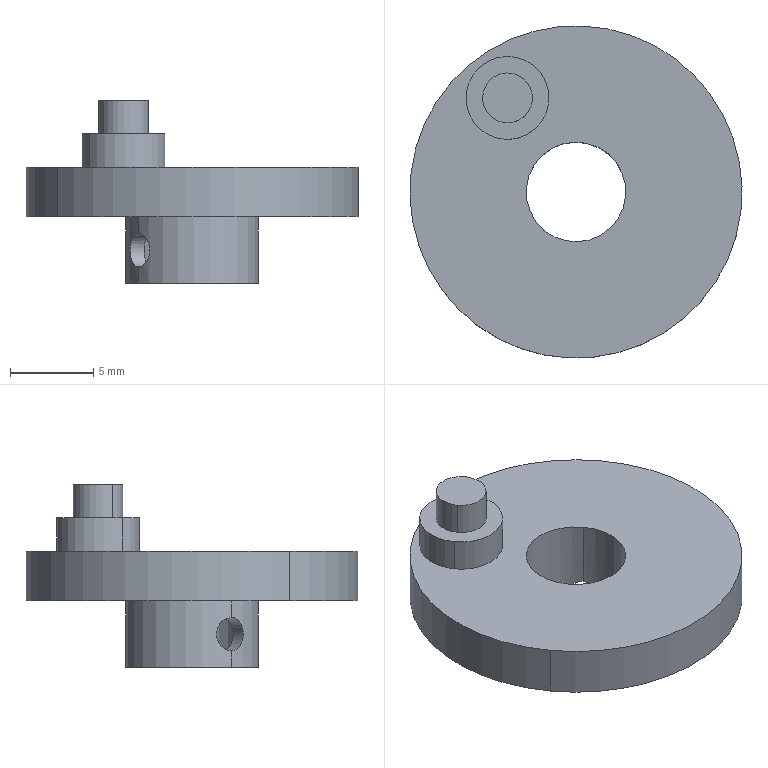Component | SolidWorks | 10-1 | 1 solid | 19 faces | box 20 x 20 x 11 mm | volume 993 mm3 | cylinder 14 | plane 5 | commonest cylinder face diameters 2 x4 8 x2 6 x2 3 x2 5 x2 20 x2
build123d program:
from build123d import *

# Parameters (mm, degrees)
SKETCH1_R           = 10
BOSS_EXTRUDE1_DEPTH = 3
SKETCH2_R           = 2.5
BOSS_EXTRUDE2_DEPTH = 2
SKETCH3_R           = 1.5
BOSS_EXTRUDE3_DEPTH = 2
SKETCH4_R           = 3
CUT_EXTRUDE1_DEPTH  = 24
BOSS_EXTRUDE4_START = 4
SKETCH5_R           = 4
SKETCH5_R_2         = 3
BOSS_EXTRUDE4_DEPTH = 4
SKETCH6_R           = 1
CUT_EXTRUDE2_DEPTH  = 5


with BuildPart() as part:
    # Sketch1 → Boss-Extrude1 (new body)
    with BuildSketch(Plane.XY):
        Circle(SKETCH1_R)
    extrude(amount=BOSS_EXTRUDE1_DEPTH)

    # Sketch2 → Boss-Extrude2 (add)
    with BuildSketch(Plane.XY.offset(3)):
        with Locations((0, 7)):
            Circle(SKETCH2_R)
    extrude(amount=BOSS_EXTRUDE2_DEPTH)

    # Sketch3 → Boss-Extrude3 (add)
    with BuildSketch(Plane.XY.offset(5)):
        with Locations((0, 7)):
            Circle(SKETCH3_R)
    extrude(amount=BOSS_EXTRUDE3_DEPTH)

    # Sketch4 → Cut-Extrude1 (cut)
    with BuildSketch(Plane(origin=(0, 0, 0), x_dir=(-1, 0, 0), z_dir=(0, 0, -1))):
        Circle(SKETCH4_R)
    extrude(amount=-CUT_EXTRUDE1_DEPTH, mode=Mode.SUBTRACT)

    # Sketch5 → Boss-Extrude4 (add)
    with BuildSketch(Plane(origin=(0, 0, 0), x_dir=(-1, 0, 0), z_dir=(0, 0, -1)).offset(BOSS_EXTRUDE4_START)):
        with Locations(Location((0, 0, 0), (0, 0, 180))):
            Circle(SKETCH5_R)
        Circle(SKETCH5_R_2, mode=Mode.SUBTRACT)
    extrude(amount=-BOSS_EXTRUDE4_DEPTH)

    # Sketch6 → Cut-Extrude2 (cut, symmetric)
    with BuildSketch(Plane(origin=(0, 0, 0), x_dir=(0, 0, -1), z_dir=(1, 0, 0))):
        with Locations((2, 0)):
            Circle(SKETCH6_R)
    extrude(amount=CUT_EXTRUDE2_DEPTH, both=True, mode=Mode.SUBTRACT)


solid = part.part

# Placed as in the assembly
solid = solid.moved(Location((69.329, 7.034, 22.938), (0, 0, 36.07)))
STEP:
#1=COLOUR_RGB('',0.7922,0.8196,0.9333);
#2=FILL_AREA_STYLE_COLOUR('',#1);
#3=FILL_AREA_STYLE('',(#2));
#4=SURFACE_STYLE_FILL_AREA(#3);
#5=SURFACE_SIDE_STYLE('',(#4));
#6=SURFACE_STYLE_USAGE(.BOTH.,#5);
#7=PRESENTATION_STYLE_ASSIGNMENT((#6));
#8=CARTESIAN_POINT('',(2.825,0.3465,0.8637));
#9=VERTEX_POINT('',#8);
#10=CARTESIAN_POINT('',(2.825,0.3465,0.785));
#11=VERTEX_POINT('',#10);
#12=CARTESIAN_POINT('',(2.825,0.3465,0.8637));
#13=CARTESIAN_POINT('',(2.828,0.3423,0.8637));
#14=CARTESIAN_POINT('',(2.831,0.3379,0.8627));
#15=CARTESIAN_POINT('',(2.835,0.3295,0.8587));
#16=CARTESIAN_POINT('',(2.837,0.3255,0.8558));
#17=CARTESIAN_POINT('',(2.84,0.3185,0.8485));
#18=CARTESIAN_POINT('',(2.841,0.3157,0.8442));
#19=CARTESIAN_POINT('',(2.842,0.3117,0.8347));
#20=CARTESIAN_POINT('',(2.843,0.3107,0.8295));
#21=CARTESIAN_POINT('',(2.843,0.3107,0.8191));
#22=CARTESIAN_POINT('',(2.842,0.3117,0.8139));
#23=CARTESIAN_POINT('',(2.841,0.3157,0.8045));
#24=CARTESIAN_POINT('',(2.84,0.3186,0.8001));
#25=CARTESIAN_POINT('',(2.837,0.3254,0.7929));
#26=CARTESIAN_POINT('',(2.835,0.3294,0.79));
#27=CARTESIAN_POINT('',(2.831,0.3379,0.786));
#28=CARTESIAN_POINT('',(2.828,0.3422,0.785));
#29=CARTESIAN_POINT('',(2.825,0.3465,0.785));
#30=B_SPLINE_CURVE_WITH_KNOTS('',3,(#12,#13,#14,#15,#16,#17,#18,#19,#20,#21,#22,#23,#24,#25,#26,#27,#28,#29),.UNSPECIFIED.,.F.,.F.,(4,2,2,2,2,2,2,2,4),(0.003149,0.003543,0.003936,0.00433,0.004723,0.005117,0.00551,0.005904,0.006298),.UNSPECIFIED.);
#31=EDGE_CURVE('',#9,#11,#30,.T.);
#32=ORIENTED_EDGE('',*,*,#31,.F.);
#33=CARTESIAN_POINT('',(2.857,0.3696,0.8637));
#34=VERTEX_POINT('',#33);
#35=CARTESIAN_POINT('',(2.57,0.161,0.8637));
#36=DIRECTION('',(0.8083,0.5888,-0.));
#37=VECTOR('',#36,39.37);
#38=LINE('',#35,#37);
#39=EDGE_CURVE('',#9,#34,#38,.T.);
#40=ORIENTED_EDGE('',*,*,#39,.T.);
#41=CARTESIAN_POINT('',(2.857,0.3696,0.785));
#42=VERTEX_POINT('',#41);
#43=CARTESIAN_POINT('',(2.857,0.3696,0.785));
#44=CARTESIAN_POINT('',(2.86,0.3654,0.785));
#45=CARTESIAN_POINT('',(2.863,0.3611,0.786));
#46=CARTESIAN_POINT('',(2.868,0.3529,0.79));
#47=CARTESIAN_POINT('',(2.87,0.349,0.7929));
#48=CARTESIAN_POINT('',(2.873,0.3424,0.8001));
#49=CARTESIAN_POINT('',(2.874,0.3396,0.8045));
#50=CARTESIAN_POINT('',(2.876,0.3359,0.814));
#51=CARTESIAN_POINT('',(2.876,0.3349,0.8192));
#52=CARTESIAN_POINT('',(2.876,0.3349,0.8295));
#53=CARTESIAN_POINT('',(2.876,0.3359,0.8346));
#54=CARTESIAN_POINT('',(2.874,0.3396,0.8442));
#55=CARTESIAN_POINT('',(2.873,0.3424,0.8485));
#56=CARTESIAN_POINT('',(2.87,0.349,0.8558));
#57=CARTESIAN_POINT('',(2.868,0.3529,0.8587));
#58=CARTESIAN_POINT('',(2.863,0.3611,0.8627));
#59=CARTESIAN_POINT('',(2.86,0.3655,0.8637));
#60=CARTESIAN_POINT('',(2.857,0.3696,0.8637));
#61=B_SPLINE_CURVE_WITH_KNOTS('',3,(#43,#44,#45,#46,#47,#48,#49,#50,#51,#52,#53,#54,#55,#56,#57,#58,#59,#60),.UNSPECIFIED.,.F.,.F.,(4,2,2,2,2,2,2,2,4),(0.,0.0003924,0.0007847,0.001177,0.001569,0.001962,0.002354,0.002747,0.003139),.UNSPECIFIED.);
#62=EDGE_CURVE('',#42,#34,#61,.T.);
#63=ORIENTED_EDGE('',*,*,#62,.F.);
#64=CARTESIAN_POINT('',(2.57,0.161,0.785));
#65=DIRECTION('',(0.8083,0.5888,-0.));
#66=VECTOR('',#65,39.37);
#67=LINE('',#64,#66);
#68=EDGE_CURVE('',#11,#42,#67,.T.);
#69=ORIENTED_EDGE('',*,*,#68,.F.);
#70=EDGE_LOOP('',(#32,#40,#63,#69));
#71=FACE_OUTER_BOUND('',#70,.T.);
#72=CARTESIAN_POINT('',(2.57,0.161,0.8243));
#73=DIRECTION('',(0.8083,0.5888,-0.));
#74=DIRECTION('',(0.,-0.,-1.));
#75=AXIS2_PLACEMENT_3D('',#72,#73,#74);
#76=CYLINDRICAL_SURFACE('',#75,0.03937);
#77=ADVANCED_FACE('',(#71),#76,.F.);
#78=CARTESIAN_POINT('',(2.602,0.1842,0.8637));
#79=VERTEX_POINT('',#78);
#80=CARTESIAN_POINT('',(2.602,0.1842,0.785));
#81=VERTEX_POINT('',#80);
#82=CARTESIAN_POINT('',(2.602,0.1842,0.8637));
#83=CARTESIAN_POINT('',(2.605,0.18,0.8637));
#84=CARTESIAN_POINT('',(2.609,0.176,0.8627));
#85=CARTESIAN_POINT('',(2.615,0.1689,0.8587));
#86=CARTESIAN_POINT('',(2.618,0.1657,0.8558));
#87=CARTESIAN_POINT('',(2.623,0.1606,0.8486));
#88=CARTESIAN_POINT('',(2.626,0.1587,0.8442));
#89=CARTESIAN_POINT('',(2.629,0.156,0.8347));
#90=CARTESIAN_POINT('',(2.629,0.1553,0.8295));
#91=CARTESIAN_POINT('',(2.629,0.1553,0.8192));
#92=CARTESIAN_POINT('',(2.629,0.156,0.814));
#93=CARTESIAN_POINT('',(2.626,0.1586,0.8045));
#94=CARTESIAN_POINT('',(2.623,0.1606,0.8001));
#95=CARTESIAN_POINT('',(2.618,0.1657,0.7929));
#96=CARTESIAN_POINT('',(2.615,0.1688,0.79));
#97=CARTESIAN_POINT('',(2.609,0.176,0.786));
#98=CARTESIAN_POINT('',(2.605,0.18,0.785));
#99=CARTESIAN_POINT('',(2.602,0.1842,0.785));
#100=B_SPLINE_CURVE_WITH_KNOTS('',3,(#82,#83,#84,#85,#86,#87,#88,#89,#90,#91,#92,#93,#94,#95,#96,#97,#98,#99),.UNSPECIFIED.,.F.,.F.,(4,2,2,2,2,2,2,2,4),(0.003139,0.003531,0.003923,0.004316,0.004708,0.0051,0.005493,0.005885,0.006277),.UNSPECIFIED.);
#101=EDGE_CURVE('',#79,#81,#100,.T.);
#102=ORIENTED_EDGE('',*,*,#101,.F.);
#103=CARTESIAN_POINT('',(2.634,0.2074,0.8637));
#104=VERTEX_POINT('',#103);
#105=CARTESIAN_POINT('',(2.57,0.161,0.8637));
#106=DIRECTION('',(0.8083,0.5888,-0.));
#107=VECTOR('',#106,39.37);
#108=LINE('',#105,#107);
#109=EDGE_CURVE('',#79,#104,#108,.T.);
#110=ORIENTED_EDGE('',*,*,#109,.T.);
#111=CARTESIAN_POINT('',(2.634,0.2074,0.785));
#112=VERTEX_POINT('',#111);
#113=CARTESIAN_POINT('',(2.634,0.2074,0.785));
#114=CARTESIAN_POINT('',(2.637,0.2032,0.785));
#115=CARTESIAN_POINT('',(2.64,0.1992,0.786));
#116=CARTESIAN_POINT('',(2.647,0.1923,0.79));
#117=CARTESIAN_POINT('',(2.65,0.1893,0.7929));
#118=CARTESIAN_POINT('',(2.656,0.1844,0.8001));
#119=CARTESIAN_POINT('',(2.658,0.1826,0.8044));
#120=CARTESIAN_POINT('',(2.662,0.1802,0.814));
#121=CARTESIAN_POINT('',(2.663,0.1795,0.8192));
#122=CARTESIAN_POINT('',(2.663,0.1795,0.8295));
#123=CARTESIAN_POINT('',(2.662,0.1802,0.8347));
#124=CARTESIAN_POINT('',(2.658,0.1826,0.8442));
#125=CARTESIAN_POINT('',(2.656,0.1844,0.8486));
#126=CARTESIAN_POINT('',(2.65,0.1892,0.8558));
#127=CARTESIAN_POINT('',(2.647,0.1922,0.8587));
#128=CARTESIAN_POINT('',(2.64,0.1992,0.8627));
#129=CARTESIAN_POINT('',(2.637,0.2032,0.8637));
#130=CARTESIAN_POINT('',(2.634,0.2074,0.8637));
#131=B_SPLINE_CURVE_WITH_KNOTS('',3,(#113,#114,#115,#116,#117,#118,#119,#120,#121,#122,#123,#124,#125,#126,#127,#128,#129,#130),.UNSPECIFIED.,.F.,.F.,(4,2,2,2,2,2,2,2,4),(0.003149,0.003543,0.003936,0.00433,0.004723,0.005117,0.00551,0.005904,0.006298),.UNSPECIFIED.);
#132=EDGE_CURVE('',#112,#104,#131,.T.);
#133=ORIENTED_EDGE('',*,*,#132,.F.);
#134=CARTESIAN_POINT('',(2.57,0.161,0.785));
#135=DIRECTION('',(0.8083,0.5888,-0.));
#136=VECTOR('',#135,39.37);
#137=LINE('',#134,#136);
#138=EDGE_CURVE('',#81,#112,#137,.T.);
#139=ORIENTED_EDGE('',*,*,#138,.F.);
#140=EDGE_LOOP('',(#102,#110,#133,#139));
#141=FACE_OUTER_BOUND('',#140,.T.);
#142=CARTESIAN_POINT('',(2.57,0.161,0.8243));
#143=DIRECTION('',(0.8083,0.5888,-0.));
#144=DIRECTION('',(0.,-0.,-1.));
#145=AXIS2_PLACEMENT_3D('',#142,#143,#144);
#146=CYLINDRICAL_SURFACE('',#145,0.03937);
#147=ADVANCED_FACE('',(#141),#146,.F.);
#148=CARTESIAN_POINT('',(2.602,0.1842,0.7456));
#149=VERTEX_POINT('',#148);
#150=CARTESIAN_POINT('',(2.857,0.3696,0.7456));
#151=VERTEX_POINT('',#150);
#152=CARTESIAN_POINT('',(2.73,0.2769,0.7456));
#153=DIRECTION('',(-0.,-0.,-1.));
#154=DIRECTION('',(-0.8083,-0.5888,0.));
#155=AXIS2_PLACEMENT_3D('',#152,#153,#154);
#156=CIRCLE('',#155,0.1575);
#157=EDGE_CURVE('',#149,#151,#156,.T.);
#158=ORIENTED_EDGE('',*,*,#157,.F.);
#159=CARTESIAN_POINT('',(2.602,0.1842,0.7456));
#160=DIRECTION('',(0.,0.,1.));
#161=VECTOR('',#160,39.37);
#162=LINE('',#159,#161);
#163=EDGE_CURVE('',#149,#81,#162,.T.);
#164=ORIENTED_EDGE('',*,*,#163,.T.);
#165=CARTESIAN_POINT('',(2.602,0.1842,0.785));
#166=CARTESIAN_POINT('',(2.599,0.1884,0.785));
#167=CARTESIAN_POINT('',(2.596,0.1927,0.786));
#168=CARTESIAN_POINT('',(2.591,0.201,0.79));
#169=CARTESIAN_POINT('',(2.589,0.2049,0.7929));
#170=CARTESIAN_POINT('',(2.586,0.2115,0.8001));
#171=CARTESIAN_POINT('',(2.585,0.2142,0.8045));
#172=CARTESIAN_POINT('',(2.583,0.218,0.814));
#173=CARTESIAN_POINT('',(2.583,0.219,0.8192));
#174=CARTESIAN_POINT('',(2.583,0.219,0.8295));
#175=CARTESIAN_POINT('',(2.583,0.218,0.8346));
#176=CARTESIAN_POINT('',(2.585,0.2142,0.8442));
#177=CARTESIAN_POINT('',(2.586,0.2115,0.8485));
#178=CARTESIAN_POINT('',(2.589,0.2048,0.8558));
#179=CARTESIAN_POINT('',(2.591,0.2009,0.8587));
#180=CARTESIAN_POINT('',(2.596,0.1927,0.8627));
#181=CARTESIAN_POINT('',(2.599,0.1884,0.8637));
#182=CARTESIAN_POINT('',(2.602,0.1842,0.8637));
#183=B_SPLINE_CURVE_WITH_KNOTS('',3,(#165,#166,#167,#168,#169,#170,#171,#172,#173,#174,#175,#176,#177,#178,#179,#180,#181,#182),.UNSPECIFIED.,.F.,.F.,(4,2,2,2,2,2,2,2,4),(0.,0.0003924,0.0007847,0.001177,0.001569,0.001962,0.002354,0.002747,0.003139),.UNSPECIFIED.);
#184=EDGE_CURVE('',#81,#79,#183,.T.);
#185=ORIENTED_EDGE('',*,*,#184,.T.);
#186=CARTESIAN_POINT('',(2.602,0.1842,0.9031));
#187=VERTEX_POINT('',#186);
#188=CARTESIAN_POINT('',(2.602,0.1842,0.7456));
#189=DIRECTION('',(0.,0.,1.));
#190=VECTOR('',#189,39.37);
#191=LINE('',#188,#190);
#192=EDGE_CURVE('',#79,#187,#191,.T.);
#193=ORIENTED_EDGE('',*,*,#192,.T.);
#194=CARTESIAN_POINT('',(2.857,0.3696,0.9031));
#195=VERTEX_POINT('',#194);
#196=CARTESIAN_POINT('',(2.73,0.2769,0.9031));
#197=DIRECTION('',(-0.,-0.,-1.));
#198=DIRECTION('',(0.8083,0.5888,-0.));
#199=AXIS2_PLACEMENT_3D('',#196,#197,#198);
#200=CIRCLE('',#199,0.1575);
#201=EDGE_CURVE('',#187,#195,#200,.T.);
#202=ORIENTED_EDGE('',*,*,#201,.T.);
#203=CARTESIAN_POINT('',(2.857,0.3696,0.7456));
#204=DIRECTION('',(0.,0.,1.));
#205=VECTOR('',#204,39.37);
#206=LINE('',#203,#205);
#207=EDGE_CURVE('',#34,#195,#206,.T.);
#208=ORIENTED_EDGE('',*,*,#207,.F.);
#209=CARTESIAN_POINT('',(2.857,0.3696,0.8637));
#210=CARTESIAN_POINT('',(2.854,0.3738,0.8637));
#211=CARTESIAN_POINT('',(2.85,0.3779,0.8627));
#212=CARTESIAN_POINT('',(2.844,0.385,0.8587));
#213=CARTESIAN_POINT('',(2.841,0.3881,0.8558));
#214=CARTESIAN_POINT('',(2.836,0.3932,0.8486));
#215=CARTESIAN_POINT('',(2.834,0.3952,0.8442));
#216=CARTESIAN_POINT('',(2.83,0.3979,0.8347));
#217=CARTESIAN_POINT('',(2.83,0.3985,0.8295));
#218=CARTESIAN_POINT('',(2.83,0.3985,0.8192));
#219=CARTESIAN_POINT('',(2.83,0.3979,0.814));
#220=CARTESIAN_POINT('',(2.833,0.3952,0.8045));
#221=CARTESIAN_POINT('',(2.836,0.3932,0.8001));
#222=CARTESIAN_POINT('',(2.841,0.3882,0.7929));
#223=CARTESIAN_POINT('',(2.844,0.385,0.79));
#224=CARTESIAN_POINT('',(2.85,0.3779,0.786));
#225=CARTESIAN_POINT('',(2.854,0.3739,0.785));
#226=CARTESIAN_POINT('',(2.857,0.3696,0.785));
#227=B_SPLINE_CURVE_WITH_KNOTS('',3,(#209,#210,#211,#212,#213,#214,#215,#216,#217,#218,#219,#220,#221,#222,#223,#224,#225,#226),.UNSPECIFIED.,.F.,.F.,(4,2,2,2,2,2,2,2,4),(0.003139,0.003531,0.003923,0.004316,0.004708,0.0051,0.005493,0.005885,0.006277),.UNSPECIFIED.);
#228=EDGE_CURVE('',#34,#42,#227,.T.);
#229=ORIENTED_EDGE('',*,*,#228,.T.);
#230=CARTESIAN_POINT('',(2.857,0.3696,0.7456));
#231=DIRECTION('',(0.,0.,1.));
#232=VECTOR('',#231,39.37);
#233=LINE('',#230,#232);
#234=EDGE_CURVE('',#151,#42,#233,.T.);
#235=ORIENTED_EDGE('',*,*,#234,.F.);
#236=EDGE_LOOP('',(#158,#164,#185,#193,#202,#208,#229,#235));
#237=FACE_OUTER_BOUND('',#236,.T.);
#238=CARTESIAN_POINT('',(2.73,0.2769,0.7456));
#239=DIRECTION('',(0.,0.,1.));
#240=DIRECTION('',(0.8083,0.5888,-0.));
#241=AXIS2_PLACEMENT_3D('',#238,#239,#240);
#242=CYLINDRICAL_SURFACE('',#241,0.1575);
#243=ADVANCED_FACE('',(#237),#242,.T.);
#244=CARTESIAN_POINT('',(2.634,0.2074,1.021));
#245=VERTEX_POINT('',#244);
#246=CARTESIAN_POINT('',(2.825,0.3465,1.021));
#247=VERTEX_POINT('',#246);
#248=CARTESIAN_POINT('',(2.73,0.2769,1.021));
#249=DIRECTION('',(0.,0.,1.));
#250=DIRECTION('',(0.8083,0.5888,-0.));
#251=AXIS2_PLACEMENT_3D('',#248,#249,#250);
#252=CIRCLE('',#251,0.1181);
#253=EDGE_CURVE('',#245,#247,#252,.T.);
#254=ORIENTED_EDGE('',*,*,#253,.T.);
#255=CARTESIAN_POINT('',(2.825,0.3465,1.848));
#256=DIRECTION('',(-0.,-0.,-1.));
#257=VECTOR('',#256,39.37);
#258=LINE('',#255,#257);
#259=EDGE_CURVE('',#247,#9,#258,.T.);
#260=ORIENTED_EDGE('',*,*,#259,.T.);
#261=ORIENTED_EDGE('',*,*,#31,.T.);
#262=CARTESIAN_POINT('',(2.825,0.3465,0.7456));
#263=VERTEX_POINT('',#262);
#264=CARTESIAN_POINT('',(2.825,0.3465,1.848));
#265=DIRECTION('',(-0.,-0.,-1.));
#266=VECTOR('',#265,39.37);
#267=LINE('',#264,#266);
#268=EDGE_CURVE('',#11,#263,#267,.T.);
#269=ORIENTED_EDGE('',*,*,#268,.T.);
#270=CARTESIAN_POINT('',(2.634,0.2074,0.7456));
#271=VERTEX_POINT('',#270);
#272=CARTESIAN_POINT('',(2.73,0.2769,0.7456));
#273=DIRECTION('',(-0.,-0.,-1.));
#274=DIRECTION('',(-0.8083,-0.5888,0.));
#275=AXIS2_PLACEMENT_3D('',#272,#273,#274);
#276=CIRCLE('',#275,0.1181);
#277=EDGE_CURVE('',#263,#271,#276,.T.);
#278=ORIENTED_EDGE('',*,*,#277,.T.);
#279=CARTESIAN_POINT('',(2.634,0.2074,1.848));
#280=DIRECTION('',(-0.,-0.,-1.));
#281=VECTOR('',#280,39.37);
#282=LINE('',#279,#281);
#283=EDGE_CURVE('',#112,#271,#282,.T.);
#284=ORIENTED_EDGE('',*,*,#283,.F.);
#285=ORIENTED_EDGE('',*,*,#132,.T.);
#286=CARTESIAN_POINT('',(2.634,0.2074,1.848));
#287=DIRECTION('',(-0.,-0.,-1.));
#288=VECTOR('',#287,39.37);
#289=LINE('',#286,#288);
#290=EDGE_CURVE('',#245,#104,#289,.T.);
#291=ORIENTED_EDGE('',*,*,#290,.F.);
#292=EDGE_LOOP('',(#254,#260,#261,#269,#278,#284,#285,#291));
#293=FACE_OUTER_BOUND('',#292,.T.);
#294=CARTESIAN_POINT('',(2.73,0.2769,1.848));
#295=DIRECTION('',(-0.,-0.,-1.));
#296=DIRECTION('',(-0.8083,-0.5888,0.));
#297=AXIS2_PLACEMENT_3D('',#294,#295,#296);
#298=CYLINDRICAL_SURFACE('',#297,0.1181);
#299=ADVANCED_FACE('',(#293),#298,.F.);
#300=CARTESIAN_POINT('',(2.615,0.5345,1.179));
#301=VERTEX_POINT('',#300);
#302=CARTESIAN_POINT('',(2.52,0.4649,1.179));
#303=VERTEX_POINT('',#302);
#304=CARTESIAN_POINT('',(2.567,0.4997,1.179));
#305=DIRECTION('',(0.,0.,1.));
#306=DIRECTION('',(0.8083,0.5888,-0.));
#307=AXIS2_PLACEMENT_3D('',#304,#305,#306);
#308=CIRCLE('',#307,0.05906);
#309=EDGE_CURVE('',#301,#303,#308,.T.);
#310=ORIENTED_EDGE('',*,*,#309,.F.);
#311=CARTESIAN_POINT('',(2.615,0.5345,1.1));
#312=VERTEX_POINT('',#311);
#313=CARTESIAN_POINT('',(2.615,0.5345,1.179));
#314=DIRECTION('',(-0.,-0.,-1.));
#315=VECTOR('',#314,39.37);
#316=LINE('',#313,#315);
#317=EDGE_CURVE('',#301,#312,#316,.T.);
#318=ORIENTED_EDGE('',*,*,#317,.T.);
#319=CARTESIAN_POINT('',(2.52,0.4649,1.1));
#320=VERTEX_POINT('',#319);
#321=CARTESIAN_POINT('',(2.567,0.4997,1.1));
#322=DIRECTION('',(0.,0.,1.));
#323=DIRECTION('',(0.8083,0.5888,-0.));
#324=AXIS2_PLACEMENT_3D('',#321,#322,#323);
#325=CIRCLE('',#324,0.05906);
#326=EDGE_CURVE('',#312,#320,#325,.T.);
#327=ORIENTED_EDGE('',*,*,#326,.T.);
#328=CARTESIAN_POINT('',(2.52,0.4649,1.179));
#329=DIRECTION('',(-0.,-0.,-1.));
#330=VECTOR('',#329,39.37);
#331=LINE('',#328,#330);
#332=EDGE_CURVE('',#303,#320,#331,.T.);
#333=ORIENTED_EDGE('',*,*,#332,.F.);
#334=EDGE_LOOP('',(#310,#318,#327,#333));
#335=FACE_OUTER_BOUND('',#334,.T.);
#336=CARTESIAN_POINT('',(2.567,0.4997,1.179));
#337=DIRECTION('',(-0.,-0.,-1.));
#338=DIRECTION('',(-0.8083,-0.5888,0.));
#339=AXIS2_PLACEMENT_3D('',#336,#337,#338);
#340=CYLINDRICAL_SURFACE('',#339,0.05906);
#341=ADVANCED_FACE('',(#335),#340,.T.);
#342=CARTESIAN_POINT('',(2.647,0.5576,1.1));
#343=VERTEX_POINT('',#342);
#344=CARTESIAN_POINT('',(2.488,0.4417,1.1));
#345=VERTEX_POINT('',#344);
#346=CARTESIAN_POINT('',(2.567,0.4997,1.1));
#347=DIRECTION('',(0.,0.,1.));
#348=DIRECTION('',(0.8083,0.5888,-0.));
#349=AXIS2_PLACEMENT_3D('',#346,#347,#348);
#350=CIRCLE('',#349,0.09843);
#351=EDGE_CURVE('',#343,#345,#350,.T.);
#352=ORIENTED_EDGE('',*,*,#351,.F.);
#353=CARTESIAN_POINT('',(2.647,0.5576,1.021));
#354=VERTEX_POINT('',#353);
#355=CARTESIAN_POINT('',(2.647,0.5576,1.1));
#356=DIRECTION('',(-0.,-0.,-1.));
#357=VECTOR('',#356,39.37);
#358=LINE('',#355,#357);
#359=EDGE_CURVE('',#343,#354,#358,.T.);
#360=ORIENTED_EDGE('',*,*,#359,.T.);
#361=CARTESIAN_POINT('',(2.488,0.4417,1.021));
#362=VERTEX_POINT('',#361);
#363=CARTESIAN_POINT('',(2.567,0.4997,1.021));
#364=DIRECTION('',(0.,0.,1.));
#365=DIRECTION('',(0.8083,0.5888,-0.));
#366=AXIS2_PLACEMENT_3D('',#363,#364,#365);
#367=CIRCLE('',#366,0.09843);
#368=EDGE_CURVE('',#354,#362,#367,.T.);
#369=ORIENTED_EDGE('',*,*,#368,.T.);
#370=CARTESIAN_POINT('',(2.488,0.4417,1.1));
#371=DIRECTION('',(-0.,-0.,-1.));
#372=VECTOR('',#371,39.37);
#373=LINE('',#370,#372);
#374=EDGE_CURVE('',#345,#362,#373,.T.);
#375=ORIENTED_EDGE('',*,*,#374,.F.);
#376=EDGE_LOOP('',(#352,#360,#369,#375));
#377=FACE_OUTER_BOUND('',#376,.T.);
#378=CARTESIAN_POINT('',(2.567,0.4997,1.1));
#379=DIRECTION('',(-0.,-0.,-1.));
#380=DIRECTION('',(-0.8083,-0.5888,0.));
#381=AXIS2_PLACEMENT_3D('',#378,#379,#380);
#382=CYLINDRICAL_SURFACE('',#381,0.09843);
#383=ADVANCED_FACE('',(#377),#382,.T.);
#384=CARTESIAN_POINT('',(3.048,0.5087,1.021));
#385=VERTEX_POINT('',#384);
#386=CARTESIAN_POINT('',(2.411,0.04513,1.021));
#387=VERTEX_POINT('',#386);
#388=CARTESIAN_POINT('',(2.73,0.2769,1.021));
#389=DIRECTION('',(0.,0.,1.));
#390=DIRECTION('',(0.8083,0.5888,-0.));
#391=AXIS2_PLACEMENT_3D('',#388,#389,#390);
#392=CIRCLE('',#391,0.3937);
#393=EDGE_CURVE('',#385,#387,#392,.T.);
#394=ORIENTED_EDGE('',*,*,#393,.F.);
#395=CARTESIAN_POINT('',(3.048,0.5087,0.9031));
#396=VERTEX_POINT('',#395);
#397=CARTESIAN_POINT('',(3.048,0.5087,1.021));
#398=DIRECTION('',(-0.,-0.,-1.));
#399=VECTOR('',#398,39.37);
#400=LINE('',#397,#399);
#401=EDGE_CURVE('',#385,#396,#400,.T.);
#402=ORIENTED_EDGE('',*,*,#401,.T.);
#403=CARTESIAN_POINT('',(2.411,0.04513,0.9031));
#404=VERTEX_POINT('',#403);
#405=CARTESIAN_POINT('',(2.73,0.2769,0.9031));
#406=DIRECTION('',(0.,0.,1.));
#407=DIRECTION('',(0.8083,0.5888,-0.));
#408=AXIS2_PLACEMENT_3D('',#405,#406,#407);
#409=CIRCLE('',#408,0.3937);
#410=EDGE_CURVE('',#396,#404,#409,.T.);
#411=ORIENTED_EDGE('',*,*,#410,.T.);
#412=CARTESIAN_POINT('',(2.411,0.04513,1.021));
#413=DIRECTION('',(-0.,-0.,-1.));
#414=VECTOR('',#413,39.37);
#415=LINE('',#412,#414);
#416=EDGE_CURVE('',#387,#404,#415,.T.);
#417=ORIENTED_EDGE('',*,*,#416,.F.);
#418=EDGE_LOOP('',(#394,#402,#411,#417));
#419=FACE_OUTER_BOUND('',#418,.T.);
#420=CARTESIAN_POINT('',(2.73,0.2769,1.021));
#421=DIRECTION('',(-0.,-0.,-1.));
#422=DIRECTION('',(-0.8083,-0.5888,0.));
#423=AXIS2_PLACEMENT_3D('',#420,#421,#422);
#424=CYLINDRICAL_SURFACE('',#423,0.3937);
#425=ADVANCED_FACE('',(#419),#424,.T.);
#426=CARTESIAN_POINT('',(2.73,0.2769,0.9031));
#427=DIRECTION('',(0.,0.,1.));
#428=DIRECTION('',(0.8083,0.5888,-0.));
#429=AXIS2_PLACEMENT_3D('',#426,#427,#428);
#430=CIRCLE('',#429,0.3937);
#431=EDGE_CURVE('',#404,#396,#430,.T.);
#432=ORIENTED_EDGE('',*,*,#431,.F.);
#433=ORIENTED_EDGE('',*,*,#410,.F.);
#434=EDGE_LOOP('',(#432,#433));
#435=FACE_OUTER_BOUND('',#434,.T.);
#436=CARTESIAN_POINT('',(2.73,0.2769,0.9031));
#437=DIRECTION('',(-0.,-0.,-1.));
#438=DIRECTION('',(0.8083,0.5888,-0.));
#439=AXIS2_PLACEMENT_3D('',#436,#437,#438);
#440=CIRCLE('',#439,0.1575);
#441=EDGE_CURVE('',#195,#187,#440,.T.);
#442=ORIENTED_EDGE('',*,*,#441,.F.);
#443=ORIENTED_EDGE('',*,*,#201,.F.);
#444=EDGE_LOOP('',(#442,#443));
#445=FACE_BOUND('',#444,.T.);
#446=CARTESIAN_POINT('',(2.73,0.2769,0.9031));
#447=DIRECTION('',(0.,0.,1.));
#448=DIRECTION('',(0.8083,0.5888,-0.));
#449=AXIS2_PLACEMENT_3D('',#446,#447,#448);
#450=PLANE('',#449);
#451=ADVANCED_FACE('',(#435,#445),#450,.F.);
#452=CARTESIAN_POINT('',(2.567,0.4997,1.1));
#453=DIRECTION('',(0.,0.,1.));
#454=DIRECTION('',(0.8083,0.5888,-0.));
#455=AXIS2_PLACEMENT_3D('',#452,#453,#454);
#456=CIRCLE('',#455,0.09843);
#457=EDGE_CURVE('',#345,#343,#456,.T.);
#458=ORIENTED_EDGE('',*,*,#457,.T.);
#459=ORIENTED_EDGE('',*,*,#351,.T.);
#460=EDGE_LOOP('',(#458,#459));
#461=FACE_OUTER_BOUND('',#460,.T.);
#462=CARTESIAN_POINT('',(2.567,0.4997,1.1));
#463=DIRECTION('',(0.,0.,1.));
#464=DIRECTION('',(0.8083,0.5888,-0.));
#465=AXIS2_PLACEMENT_3D('',#462,#463,#464);
#466=CIRCLE('',#465,0.05906);
#467=EDGE_CURVE('',#320,#312,#466,.T.);
#468=ORIENTED_EDGE('',*,*,#467,.F.);
#469=ORIENTED_EDGE('',*,*,#326,.F.);
#470=EDGE_LOOP('',(#468,#469));
#471=FACE_BOUND('',#470,.T.);
#472=CARTESIAN_POINT('',(2.567,0.4997,1.1));
#473=DIRECTION('',(0.,0.,1.));
#474=DIRECTION('',(0.8083,0.5888,-0.));
#475=AXIS2_PLACEMENT_3D('',#472,#473,#474);
#476=PLANE('',#475);
#477=ADVANCED_FACE('',(#461,#471),#476,.T.);
#478=ORIENTED_EDGE('',*,*,#253,.F.);
#479=CARTESIAN_POINT('',(2.73,0.2769,1.021));
#480=DIRECTION('',(0.,0.,1.));
#481=DIRECTION('',(0.8083,0.5888,-0.));
#482=AXIS2_PLACEMENT_3D('',#479,#480,#481);
#483=CIRCLE('',#482,0.1181);
#484=EDGE_CURVE('',#247,#245,#483,.T.);
#485=ORIENTED_EDGE('',*,*,#484,.F.);
#486=EDGE_LOOP('',(#478,#485));
#487=FACE_BOUND('',#486,.T.);
#488=CARTESIAN_POINT('',(2.73,0.2769,1.021));
#489=DIRECTION('',(0.,0.,1.));
#490=DIRECTION('',(0.8083,0.5888,-0.));
#491=AXIS2_PLACEMENT_3D('',#488,#489,#490);
#492=CIRCLE('',#491,0.3937);
#493=EDGE_CURVE('',#387,#385,#492,.T.);
#494=ORIENTED_EDGE('',*,*,#493,.T.);
#495=ORIENTED_EDGE('',*,*,#393,.T.);
#496=EDGE_LOOP('',(#494,#495));
#497=FACE_OUTER_BOUND('',#496,.T.);
#498=CARTESIAN_POINT('',(2.567,0.4997,1.021));
#499=DIRECTION('',(0.,0.,1.));
#500=DIRECTION('',(0.8083,0.5888,-0.));
#501=AXIS2_PLACEMENT_3D('',#498,#499,#500);
#502=CIRCLE('',#501,0.09843);
#503=EDGE_CURVE('',#362,#354,#502,.T.);
#504=ORIENTED_EDGE('',*,*,#503,.F.);
#505=ORIENTED_EDGE('',*,*,#368,.F.);
#506=EDGE_LOOP('',(#504,#505));
#507=FACE_BOUND('',#506,.T.);
#508=CARTESIAN_POINT('',(2.73,0.2769,1.021));
#509=DIRECTION('',(0.,0.,1.));
#510=DIRECTION('',(0.8083,0.5888,-0.));
#511=AXIS2_PLACEMENT_3D('',#508,#509,#510);
#512=PLANE('',#511);
#513=ADVANCED_FACE('',(#487,#497,#507),#512,.T.);
#514=ORIENTED_EDGE('',*,*,#401,.F.);
#515=ORIENTED_EDGE('',*,*,#493,.F.);
#516=ORIENTED_EDGE('',*,*,#416,.T.);
#517=ORIENTED_EDGE('',*,*,#431,.T.);
#518=EDGE_LOOP('',(#514,#515,#516,#517));
#519=FACE_OUTER_BOUND('',#518,.T.);
#520=CARTESIAN_POINT('',(2.73,0.2769,1.021));
#521=DIRECTION('',(-0.,-0.,-1.));
#522=DIRECTION('',(-0.8083,-0.5888,0.));
#523=AXIS2_PLACEMENT_3D('',#520,#521,#522);
#524=CYLINDRICAL_SURFACE('',#523,0.3937);
#525=ADVANCED_FACE('',(#519),#524,.T.);
#526=ORIENTED_EDGE('',*,*,#359,.F.);
#527=ORIENTED_EDGE('',*,*,#457,.F.);
#528=ORIENTED_EDGE('',*,*,#374,.T.);
#529=ORIENTED_EDGE('',*,*,#503,.T.);
#530=EDGE_LOOP('',(#526,#527,#528,#529));
#531=FACE_OUTER_BOUND('',#530,.T.);
#532=CARTESIAN_POINT('',(2.567,0.4997,1.1));
#533=DIRECTION('',(-0.,-0.,-1.));
#534=DIRECTION('',(-0.8083,-0.5888,0.));
#535=AXIS2_PLACEMENT_3D('',#532,#533,#534);
#536=CYLINDRICAL_SURFACE('',#535,0.09843);
#537=ADVANCED_FACE('',(#531),#536,.T.);
#538=ORIENTED_EDGE('',*,*,#317,.F.);
#539=CARTESIAN_POINT('',(2.567,0.4997,1.179));
#540=DIRECTION('',(0.,0.,1.));
#541=DIRECTION('',(0.8083,0.5888,-0.));
#542=AXIS2_PLACEMENT_3D('',#539,#540,#541);
#543=CIRCLE('',#542,0.05906);
#544=EDGE_CURVE('',#303,#301,#543,.T.);
#545=ORIENTED_EDGE('',*,*,#544,.F.);
#546=ORIENTED_EDGE('',*,*,#332,.T.);
#547=ORIENTED_EDGE('',*,*,#467,.T.);
#548=EDGE_LOOP('',(#538,#545,#546,#547));
#549=FACE_OUTER_BOUND('',#548,.T.);
#550=CARTESIAN_POINT('',(2.567,0.4997,1.179));
#551=DIRECTION('',(-0.,-0.,-1.));
#552=DIRECTION('',(-0.8083,-0.5888,0.));
#553=AXIS2_PLACEMENT_3D('',#550,#551,#552);
#554=CYLINDRICAL_SURFACE('',#553,0.05906);
#555=ADVANCED_FACE('',(#549),#554,.T.);
#556=ORIENTED_EDGE('',*,*,#544,.T.);
#557=ORIENTED_EDGE('',*,*,#309,.T.);
#558=EDGE_LOOP('',(#556,#557));
#559=FACE_OUTER_BOUND('',#558,.T.);
#560=CARTESIAN_POINT('',(2.567,0.4997,1.179));
#561=DIRECTION('',(0.,0.,1.));
#562=DIRECTION('',(0.8083,0.5888,-0.));
#563=AXIS2_PLACEMENT_3D('',#560,#561,#562);
#564=PLANE('',#563);
#565=ADVANCED_FACE('',(#559),#564,.T.);
#566=ORIENTED_EDGE('',*,*,#259,.F.);
#567=ORIENTED_EDGE('',*,*,#484,.T.);
#568=ORIENTED_EDGE('',*,*,#290,.T.);
#569=CARTESIAN_POINT('',(2.634,0.2074,0.8637));
#570=CARTESIAN_POINT('',(2.631,0.2116,0.8637));
#571=CARTESIAN_POINT('',(2.628,0.216,0.8627));
#572=CARTESIAN_POINT('',(2.624,0.2244,0.8587));
#573=CARTESIAN_POINT('',(2.622,0.2284,0.8558));
#574=CARTESIAN_POINT('',(2.619,0.2353,0.8486));
#575=CARTESIAN_POINT('',(2.618,0.2382,0.8442));
#576=CARTESIAN_POINT('',(2.617,0.2421,0.8347));
#577=CARTESIAN_POINT('',(2.616,0.2432,0.8295));
#578=CARTESIAN_POINT('',(2.616,0.2432,0.8192));
#579=CARTESIAN_POINT('',(2.617,0.2421,0.814));
#580=CARTESIAN_POINT('',(2.618,0.2382,0.8044));
#581=CARTESIAN_POINT('',(2.619,0.2353,0.8001));
#582=CARTESIAN_POINT('',(2.622,0.2284,0.7929));
#583=CARTESIAN_POINT('',(2.624,0.2244,0.79));
#584=CARTESIAN_POINT('',(2.628,0.216,0.786));
#585=CARTESIAN_POINT('',(2.631,0.2116,0.785));
#586=CARTESIAN_POINT('',(2.634,0.2074,0.785));
#587=B_SPLINE_CURVE_WITH_KNOTS('',3,(#569,#570,#571,#572,#573,#574,#575,#576,#577,#578,#579,#580,#581,#582,#583,#584,#585,#586),.UNSPECIFIED.,.F.,.F.,(4,2,2,2,2,2,2,2,4),(0.,0.0003936,0.0007873,0.001181,0.001575,0.001968,0.002362,0.002756,0.003149),.UNSPECIFIED.);
#588=EDGE_CURVE('',#104,#112,#587,.T.);
#589=ORIENTED_EDGE('',*,*,#588,.T.);
#590=ORIENTED_EDGE('',*,*,#283,.T.);
#591=CARTESIAN_POINT('',(2.73,0.2769,0.7456));
#592=DIRECTION('',(-0.,-0.,-1.));
#593=DIRECTION('',(-0.8083,-0.5888,0.));
#594=AXIS2_PLACEMENT_3D('',#591,#592,#593);
#595=CIRCLE('',#594,0.1181);
#596=EDGE_CURVE('',#271,#263,#595,.T.);
#597=ORIENTED_EDGE('',*,*,#596,.T.);
#598=ORIENTED_EDGE('',*,*,#268,.F.);
#599=CARTESIAN_POINT('',(2.825,0.3465,0.785));
#600=CARTESIAN_POINT('',(2.822,0.3507,0.785));
#601=CARTESIAN_POINT('',(2.819,0.3546,0.786));
#602=CARTESIAN_POINT('',(2.812,0.3616,0.79));
#603=CARTESIAN_POINT('',(2.809,0.3646,0.7929));
#604=CARTESIAN_POINT('',(2.803,0.3694,0.8001));
#605=CARTESIAN_POINT('',(2.801,0.3713,0.8045));
#606=CARTESIAN_POINT('',(2.797,0.3737,0.8139));
#607=CARTESIAN_POINT('',(2.796,0.3743,0.8191));
#608=CARTESIAN_POINT('',(2.796,0.3743,0.8295));
#609=CARTESIAN_POINT('',(2.797,0.3737,0.8347));
#610=CARTESIAN_POINT('',(2.801,0.3712,0.8443));
#611=CARTESIAN_POINT('',(2.803,0.3694,0.8486));
#612=CARTESIAN_POINT('',(2.809,0.3646,0.8558));
#613=CARTESIAN_POINT('',(2.812,0.3616,0.8587));
#614=CARTESIAN_POINT('',(2.819,0.3546,0.8627));
#615=CARTESIAN_POINT('',(2.822,0.3506,0.8637));
#616=CARTESIAN_POINT('',(2.825,0.3465,0.8637));
#617=B_SPLINE_CURVE_WITH_KNOTS('',3,(#599,#600,#601,#602,#603,#604,#605,#606,#607,#608,#609,#610,#611,#612,#613,#614,#615,#616),.UNSPECIFIED.,.F.,.F.,(4,2,2,2,2,2,2,2,4),(0.,0.0003936,0.0007873,0.001181,0.001575,0.001968,0.002362,0.002756,0.003149),.UNSPECIFIED.);
#618=EDGE_CURVE('',#11,#9,#617,.T.);
#619=ORIENTED_EDGE('',*,*,#618,.T.);
#620=EDGE_LOOP('',(#566,#567,#568,#589,#590,#597,#598,#619));
#621=FACE_OUTER_BOUND('',#620,.T.);
#622=CARTESIAN_POINT('',(2.73,0.2769,1.848));
#623=DIRECTION('',(-0.,-0.,-1.));
#624=DIRECTION('',(-0.8083,-0.5888,0.));
#625=AXIS2_PLACEMENT_3D('',#622,#623,#624);
#626=CYLINDRICAL_SURFACE('',#625,0.1181);
#627=ADVANCED_FACE('',(#621),#626,.F.);
#628=CARTESIAN_POINT('',(2.73,0.2769,0.7456));
#629=DIRECTION('',(-0.,-0.,-1.));
#630=DIRECTION('',(-0.8083,-0.5888,0.));
#631=AXIS2_PLACEMENT_3D('',#628,#629,#630);
#632=CIRCLE('',#631,0.1575);
#633=EDGE_CURVE('',#151,#149,#632,.T.);
#634=ORIENTED_EDGE('',*,*,#633,.T.);
#635=ORIENTED_EDGE('',*,*,#157,.T.);
#636=EDGE_LOOP('',(#634,#635));
#637=FACE_OUTER_BOUND('',#636,.T.);
#638=ORIENTED_EDGE('',*,*,#596,.F.);
#639=ORIENTED_EDGE('',*,*,#277,.F.);
#640=EDGE_LOOP('',(#638,#639));
#641=FACE_BOUND('',#640,.T.);
#642=CARTESIAN_POINT('',(2.73,0.2769,0.7456));
#643=DIRECTION('',(-0.,-0.,-1.));
#644=DIRECTION('',(-0.8083,-0.5888,0.));
#645=AXIS2_PLACEMENT_3D('',#642,#643,#644);
#646=PLANE('',#645);
#647=ADVANCED_FACE('',(#637,#641),#646,.T.);
#648=ORIENTED_EDGE('',*,*,#163,.F.);
#649=ORIENTED_EDGE('',*,*,#633,.F.);
#650=ORIENTED_EDGE('',*,*,#234,.T.);
#651=ORIENTED_EDGE('',*,*,#62,.T.);
#652=ORIENTED_EDGE('',*,*,#207,.T.);
#653=ORIENTED_EDGE('',*,*,#441,.T.);
#654=ORIENTED_EDGE('',*,*,#192,.F.);
#655=ORIENTED_EDGE('',*,*,#101,.T.);
#656=EDGE_LOOP('',(#648,#649,#650,#651,#652,#653,#654,#655));
#657=FACE_OUTER_BOUND('',#656,.T.);
#658=CARTESIAN_POINT('',(2.73,0.2769,0.7456));
#659=DIRECTION('',(0.,0.,1.));
#660=DIRECTION('',(0.8083,0.5888,-0.));
#661=AXIS2_PLACEMENT_3D('',#658,#659,#660);
#662=CYLINDRICAL_SURFACE('',#661,0.1575);
#663=ADVANCED_FACE('',(#657),#662,.T.);
#664=ORIENTED_EDGE('',*,*,#109,.F.);
#665=ORIENTED_EDGE('',*,*,#184,.F.);
#666=ORIENTED_EDGE('',*,*,#138,.T.);
#667=ORIENTED_EDGE('',*,*,#588,.F.);
#668=EDGE_LOOP('',(#664,#665,#666,#667));
#669=FACE_OUTER_BOUND('',#668,.T.);
#670=CARTESIAN_POINT('',(2.57,0.161,0.8243));
#671=DIRECTION('',(0.8083,0.5888,-0.));
#672=DIRECTION('',(0.,-0.,-1.));
#673=AXIS2_PLACEMENT_3D('',#670,#671,#672);
#674=CYLINDRICAL_SURFACE('',#673,0.03937);
#675=ADVANCED_FACE('',(#669),#674,.F.);
#676=ORIENTED_EDGE('',*,*,#39,.F.);
#677=ORIENTED_EDGE('',*,*,#618,.F.);
#678=ORIENTED_EDGE('',*,*,#68,.T.);
#679=ORIENTED_EDGE('',*,*,#228,.F.);
#680=EDGE_LOOP('',(#676,#677,#678,#679));
#681=FACE_OUTER_BOUND('',#680,.T.);
#682=CARTESIAN_POINT('',(2.57,0.161,0.8243));
#683=DIRECTION('',(0.8083,0.5888,-0.));
#684=DIRECTION('',(0.,-0.,-1.));
#685=AXIS2_PLACEMENT_3D('',#682,#683,#684);
#686=CYLINDRICAL_SURFACE('',#685,0.03937);
#687=ADVANCED_FACE('',(#681),#686,.F.);
#688=CLOSED_SHELL('',(#77,#147,#243,#299,#341,#383,#425,#451,#477,#513,#525,#537,#555,#565,#627,#647,#663,#675,#687));
#689=MANIFOLD_SOLID_BREP('',#688);
#690=STYLED_ITEM('',(#7),#689);
#691=PRESENTATION_LAYER_ASSIGNMENT('','',(#690));
#692=(LENGTH_UNIT()NAMED_UNIT(*)SI_UNIT($,.METRE.));
#693=LENGTH_MEASURE_WITH_UNIT(LENGTH_MEASURE(0.0254),#692);
#694=DIMENSIONAL_EXPONENTS(1.,0.,0.,0.,0.,0.,0.);
#695=(CONVERSION_BASED_UNIT('',#693)LENGTH_UNIT()NAMED_UNIT(#694));
#696=UNCERTAINTY_MEASURE_WITH_UNIT(LENGTH_MEASURE(0.00001),#695,'','');
#697=(NAMED_UNIT(*)PLANE_ANGLE_UNIT()SI_UNIT($,.RADIAN.));
#698=(NAMED_UNIT(*)SI_UNIT($,.STERADIAN.)SOLID_ANGLE_UNIT());
#699=(GEOMETRIC_REPRESENTATION_CONTEXT(3)GLOBAL_UNCERTAINTY_ASSIGNED_CONTEXT((#696))GLOBAL_UNIT_ASSIGNED_CONTEXT((#695,#697,#698))REPRESENTATION_CONTEXT('',''));
#700=MECHANICAL_DESIGN_GEOMETRIC_PRESENTATION_REPRESENTATION('',(#690),#699);
#701=CARTESIAN_POINT('',(0.,0.,0.));
#702=DIRECTION('',(0.,0.,1.));
#703=DIRECTION('',(1.,0.,0.));
#704=AXIS2_PLACEMENT_3D('',#701,#702,#703);
#705=(LENGTH_UNIT()NAMED_UNIT(*)SI_UNIT($,.METRE.));
#706=LENGTH_MEASURE_WITH_UNIT(LENGTH_MEASURE(0.0254),#705);
#707=DIMENSIONAL_EXPONENTS(1.,0.,0.,0.,0.,0.,0.);
#708=(CONVERSION_BASED_UNIT('',#706)LENGTH_UNIT()NAMED_UNIT(#707));
#709=UNCERTAINTY_MEASURE_WITH_UNIT(LENGTH_MEASURE(0.00001),#708,'','');
#710=(NAMED_UNIT(*)PLANE_ANGLE_UNIT()SI_UNIT($,.RADIAN.));
#711=(NAMED_UNIT(*)SI_UNIT($,.STERADIAN.)SOLID_ANGLE_UNIT());
#712=(GEOMETRIC_REPRESENTATION_CONTEXT(3)GLOBAL_UNCERTAINTY_ASSIGNED_CONTEXT((#709))GLOBAL_UNIT_ASSIGNED_CONTEXT((#708,#710,#711))REPRESENTATION_CONTEXT('',''));
#713=ADVANCED_BREP_SHAPE_REPRESENTATION('',(#689,#704),#712);